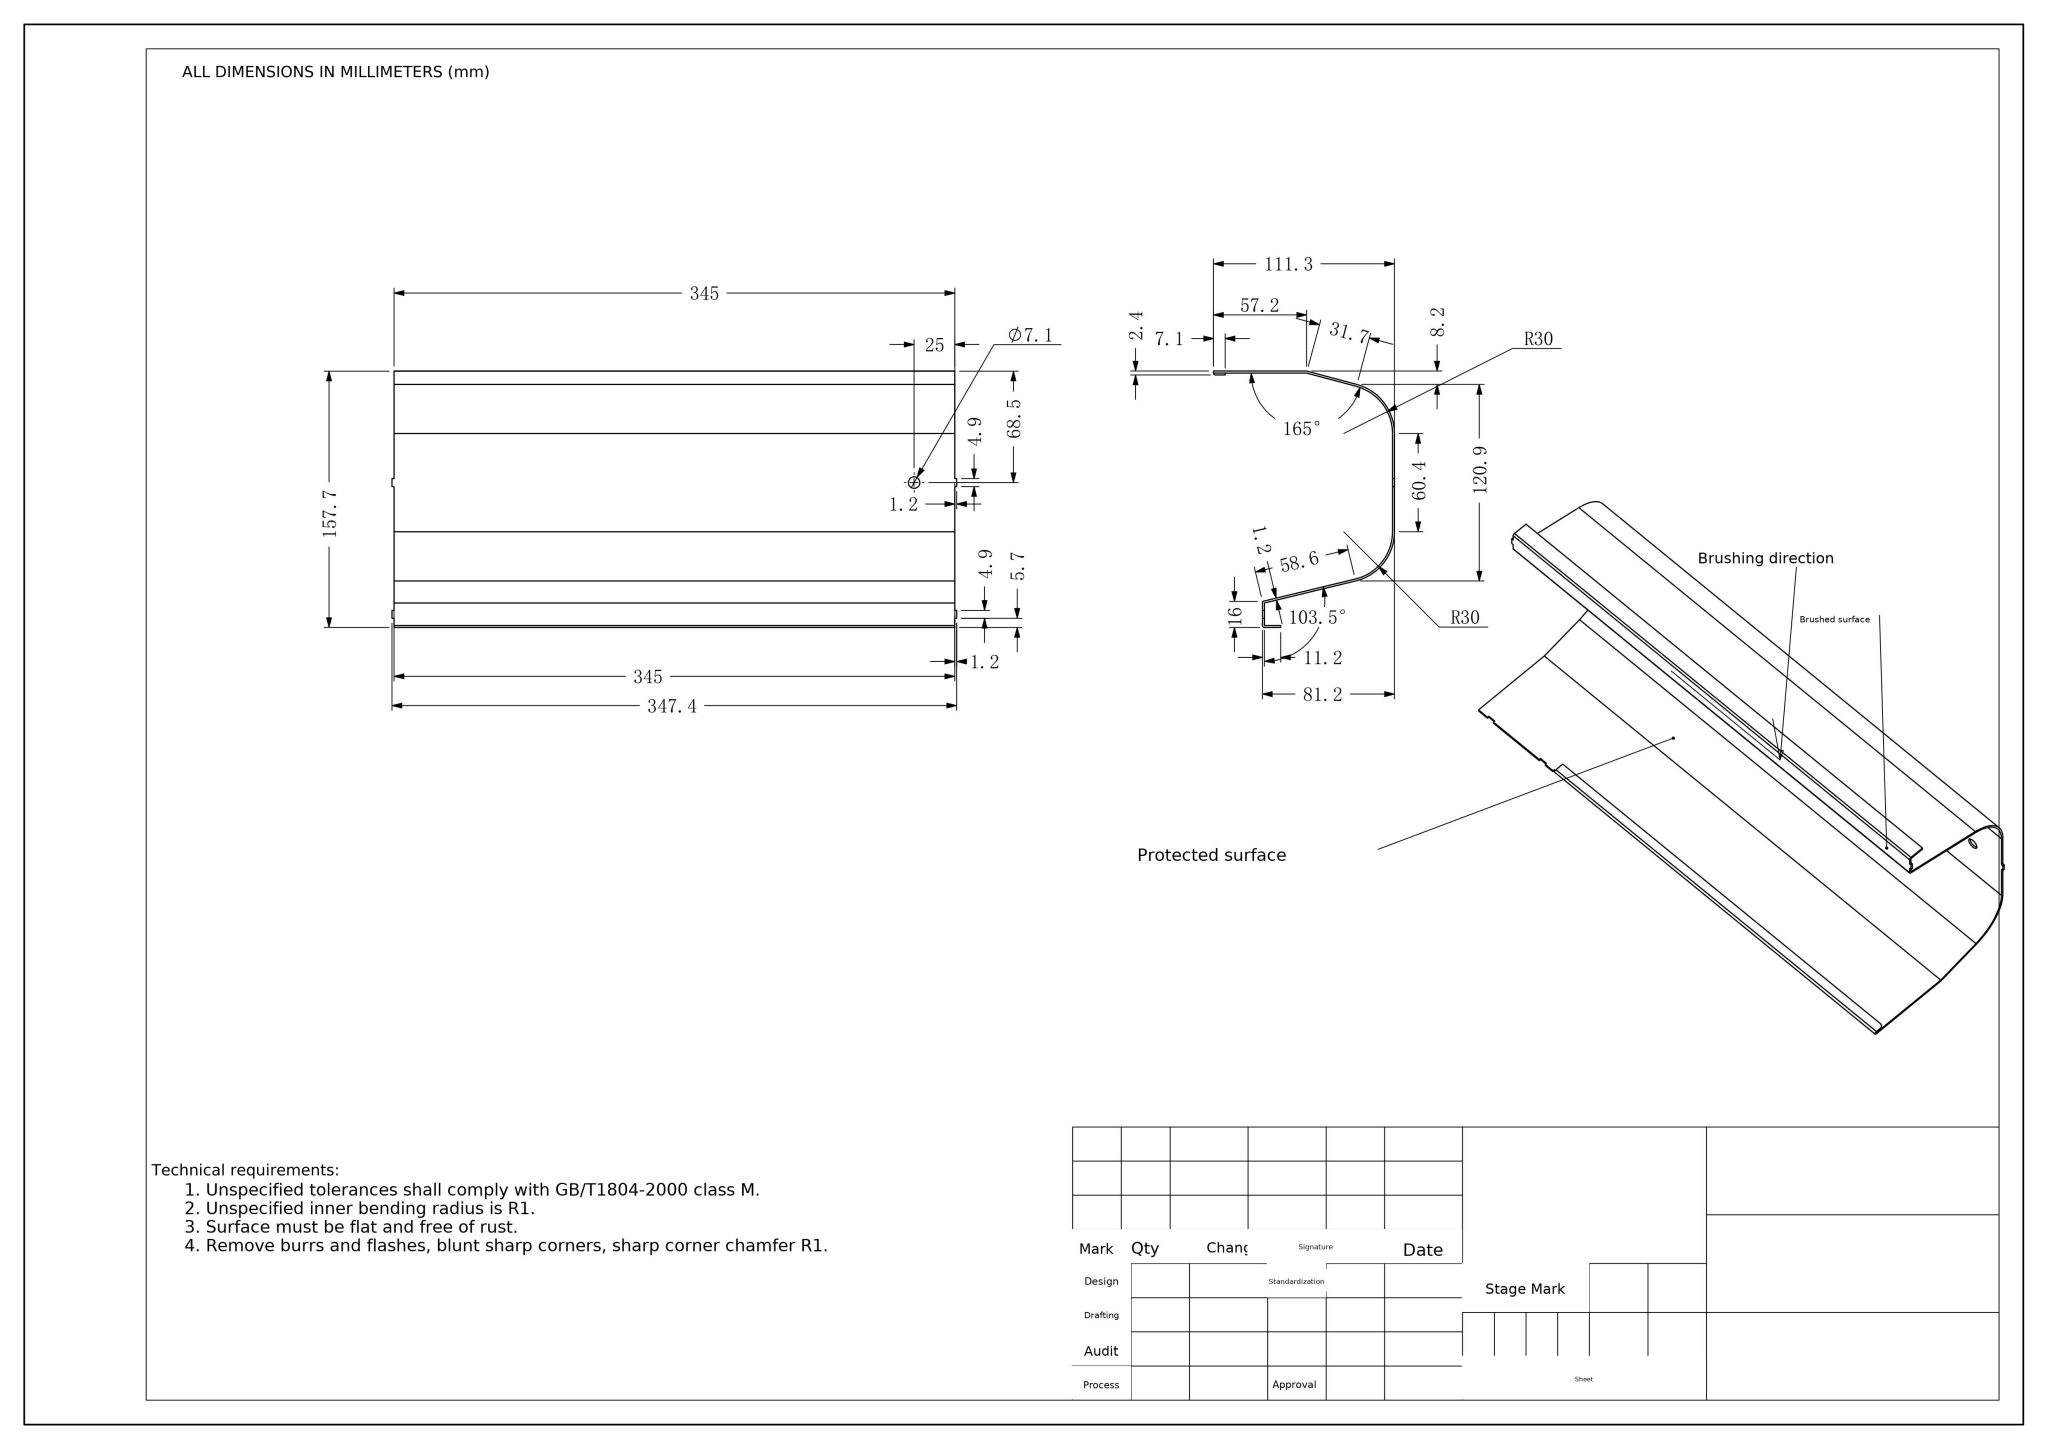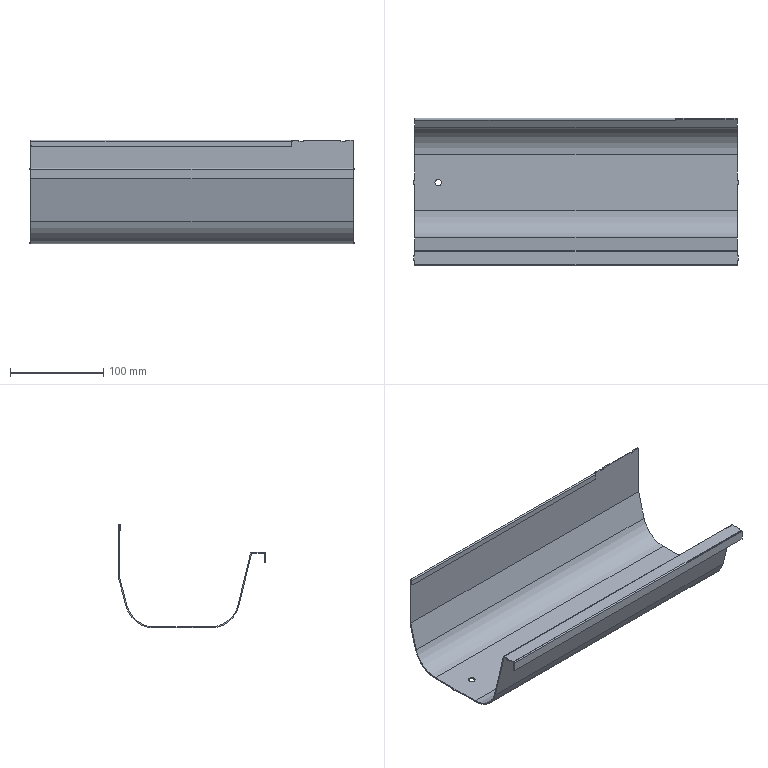Part | NX | mm | 1 solid | 62 faces | box 347.4 x 157.7 x 111.3 mm | volume 132070 mm3 | plane 46 | cylinder 16 | commonest cylinder face diameters 2.404 x3 0.004 x3 7.1 x2 60 x2 62.4 x2 0.02 x1 2.42 x1 5 x1